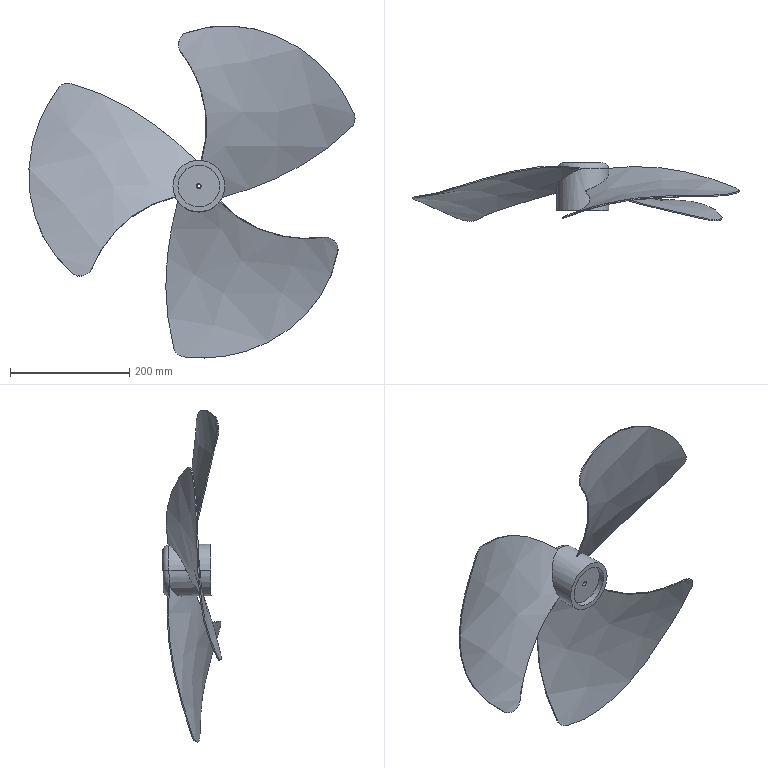Component | NX | FAN_BLADE | 2 solids | 49 faces | volume 726110 mm3 | spline 24 | cylinder 15 | plane 7 | torus 3 | commonest cylinder face diameters 86.6 x5 8 x2 70 x2 10 x2 60 x2 9.8 x1 6 x1